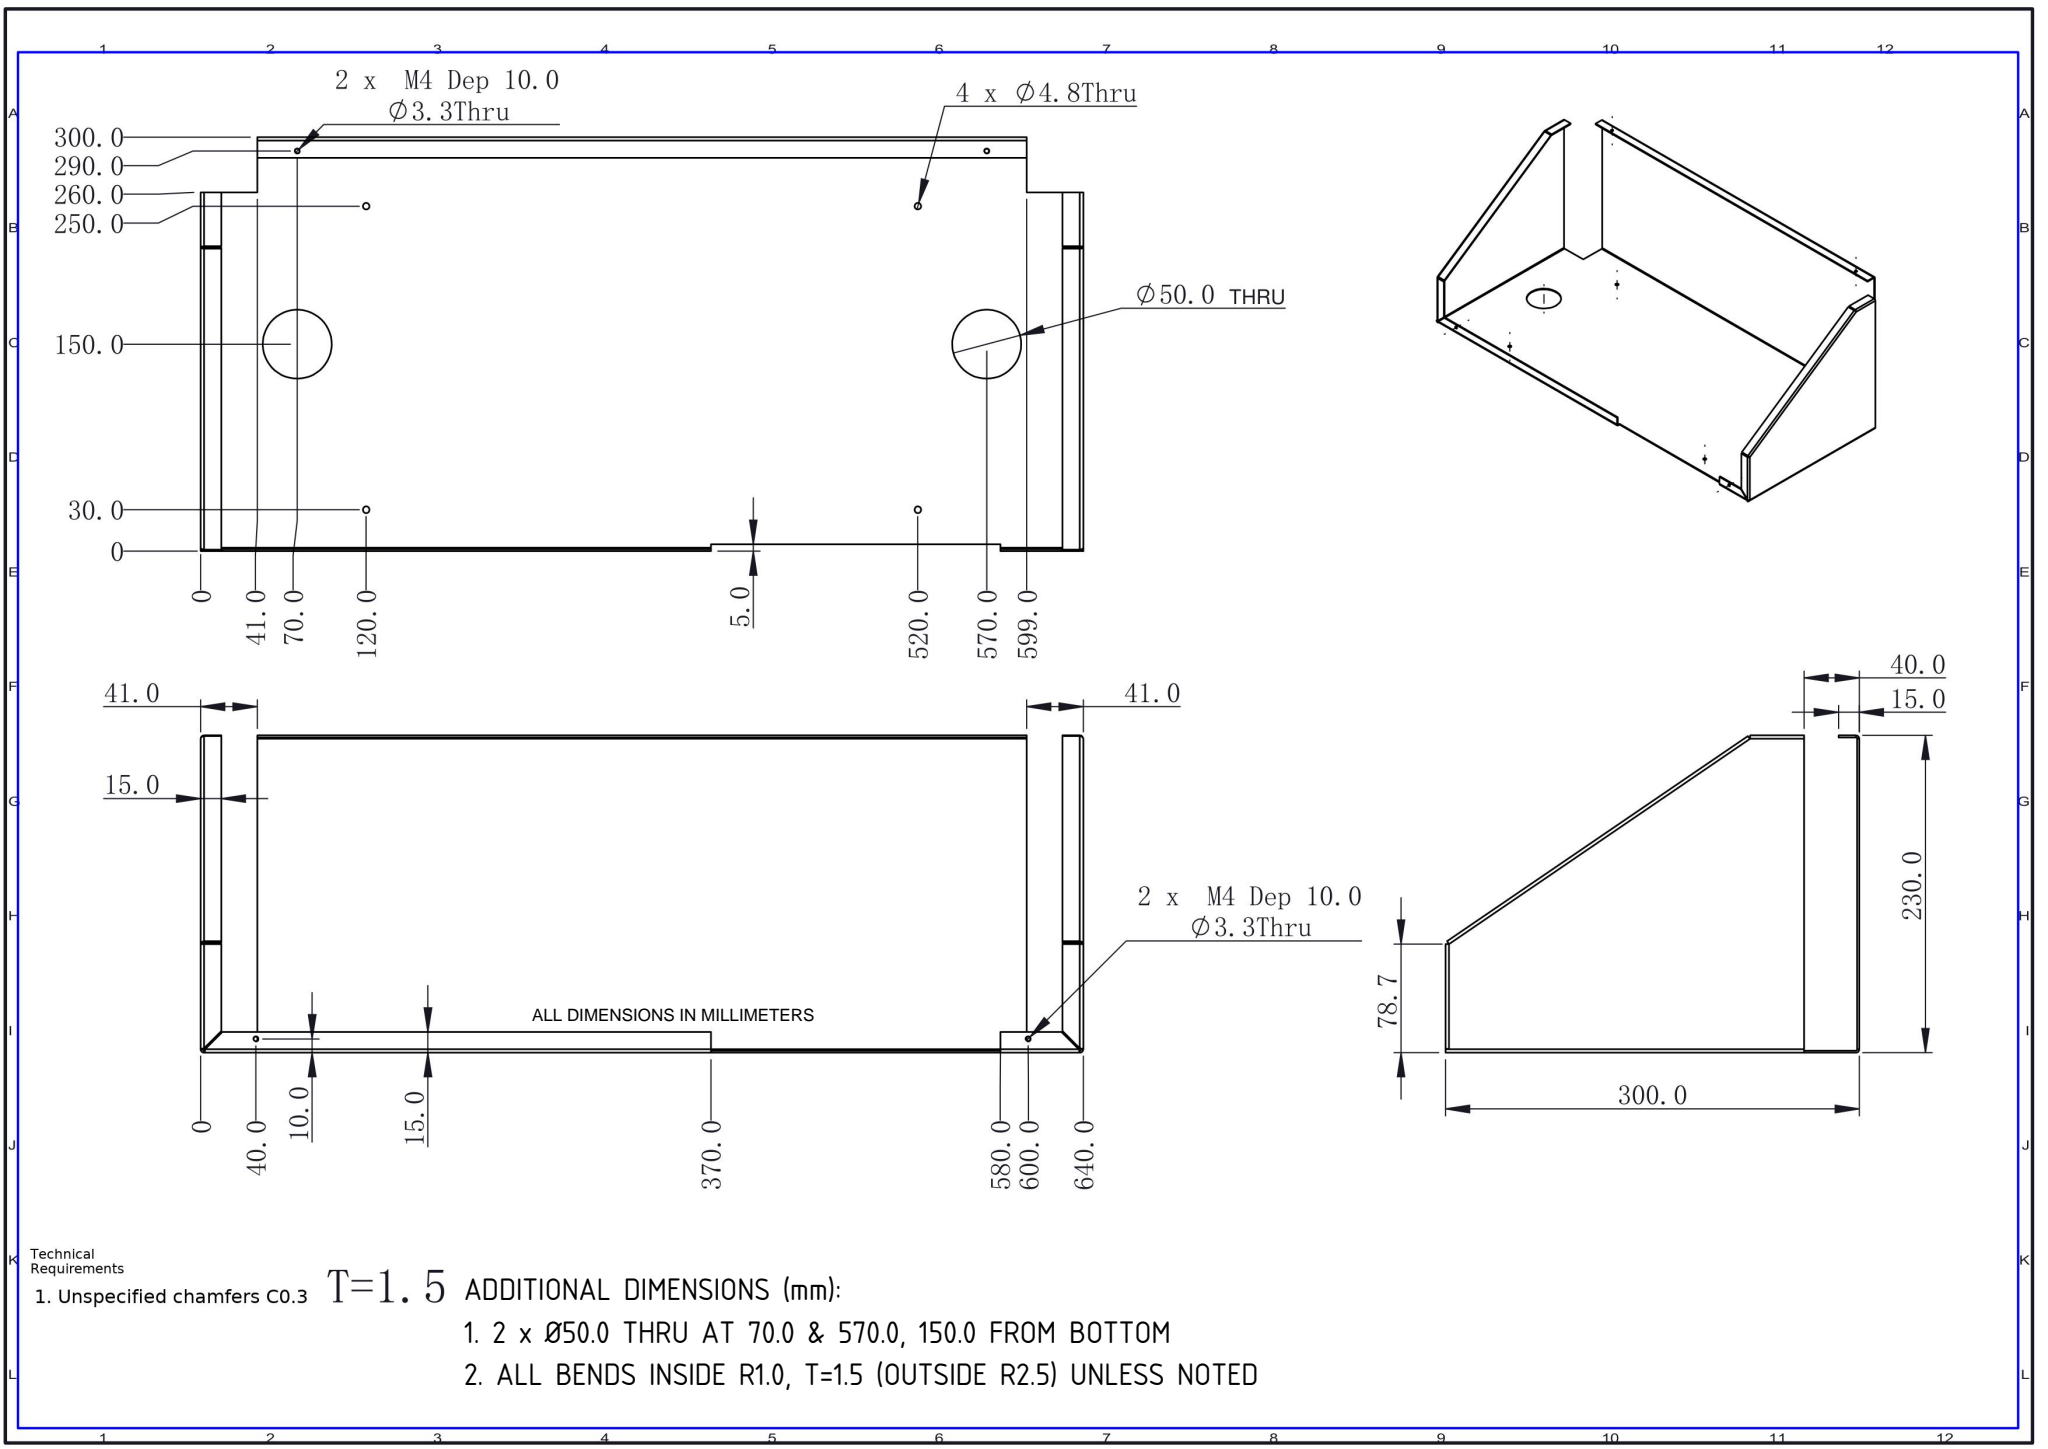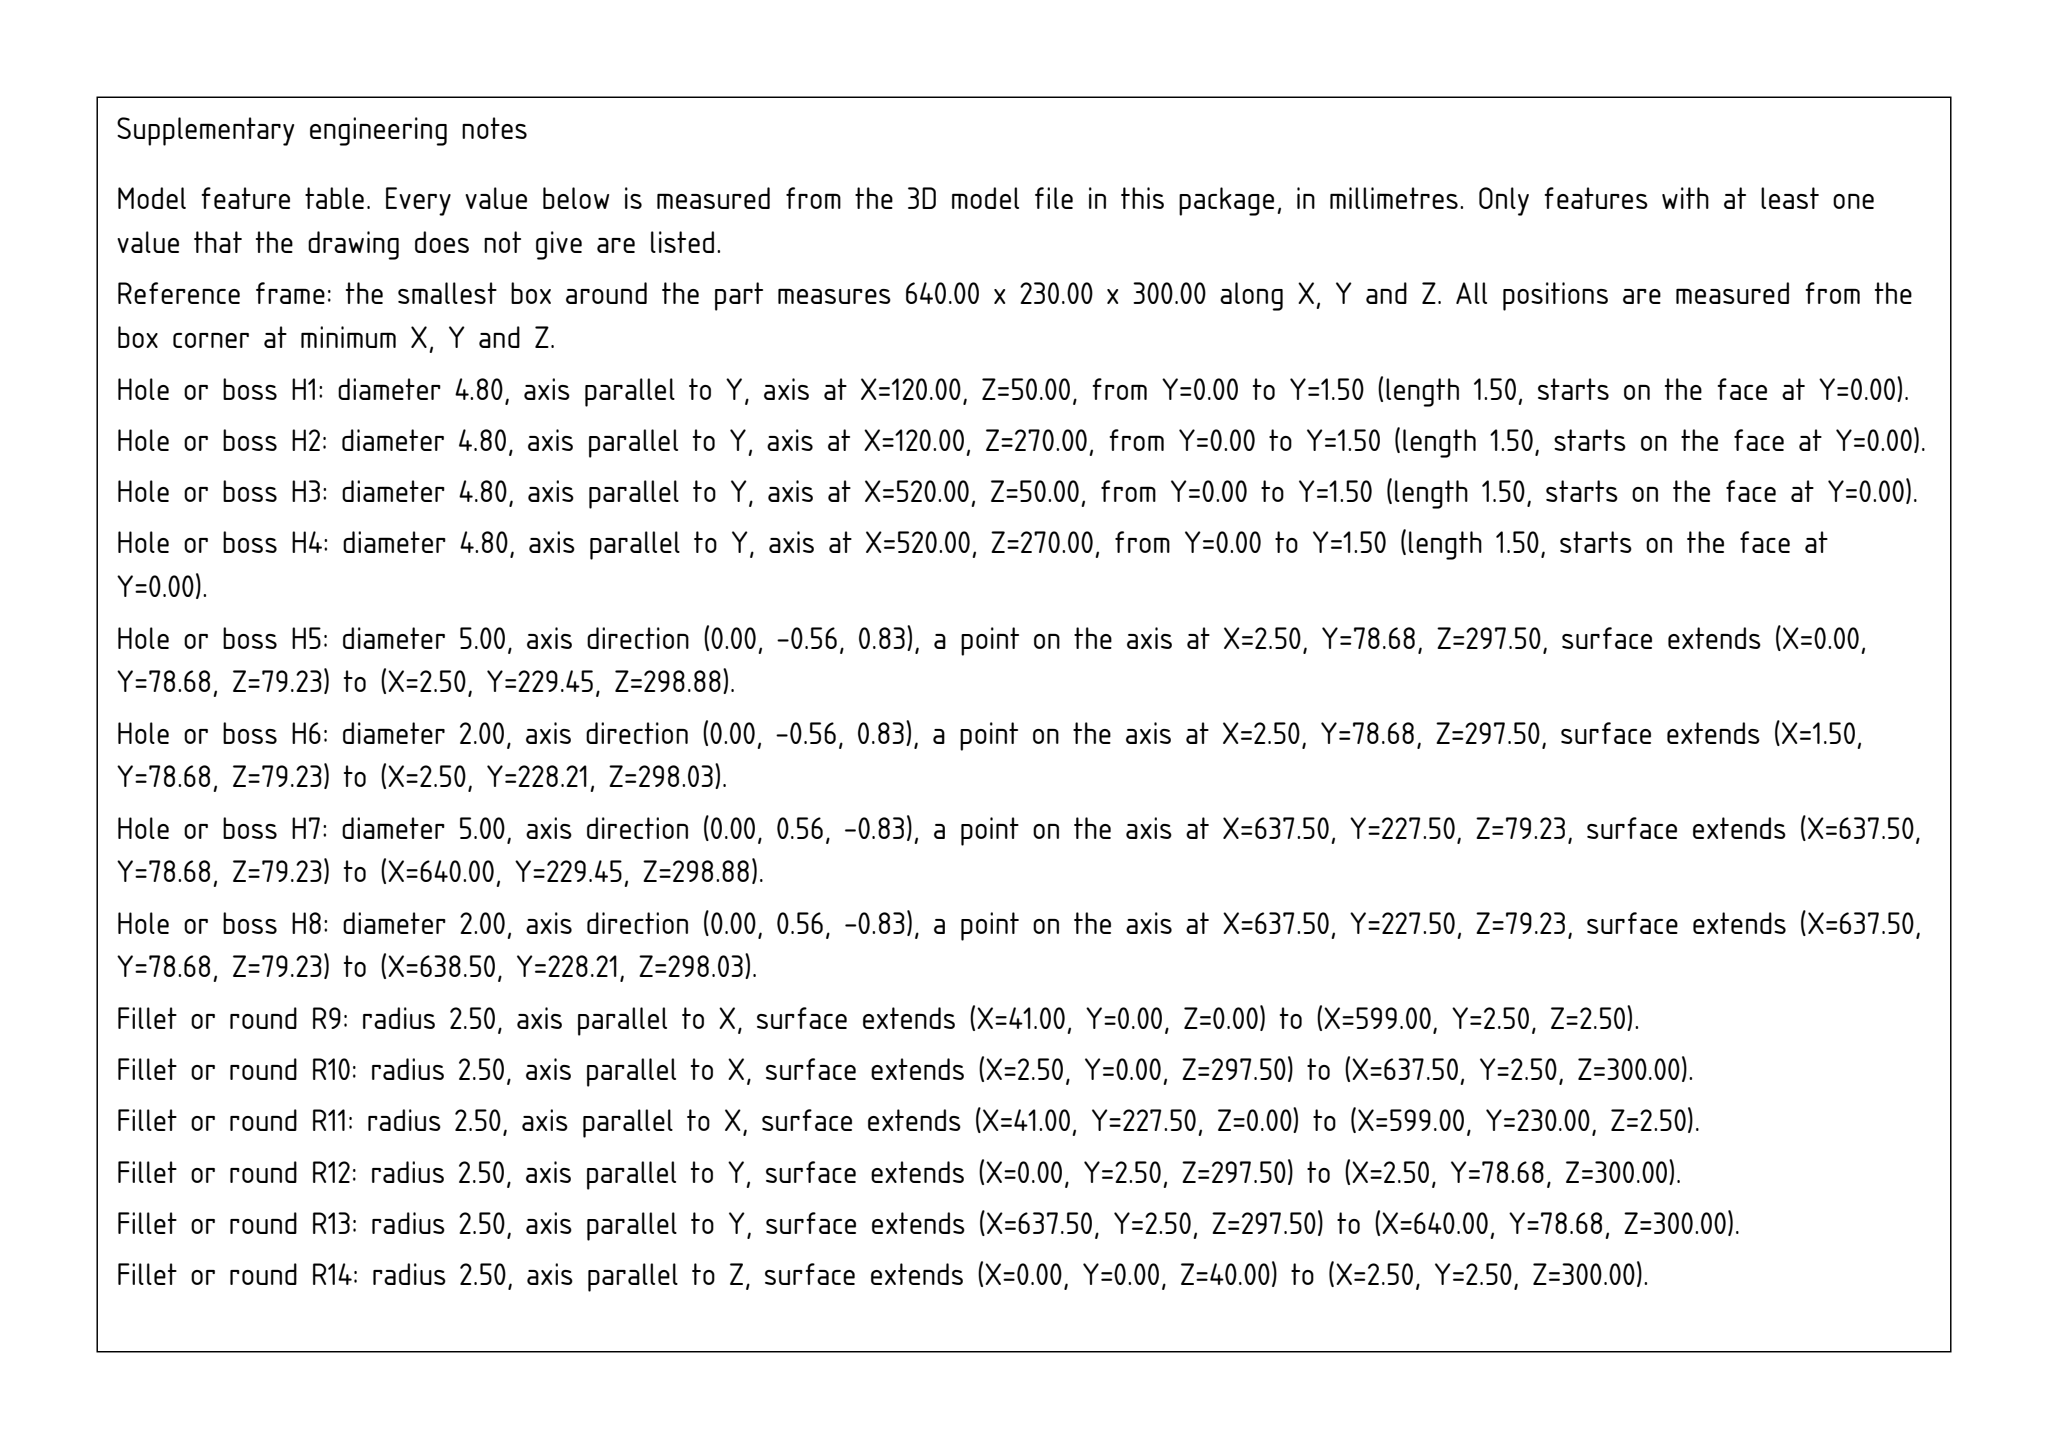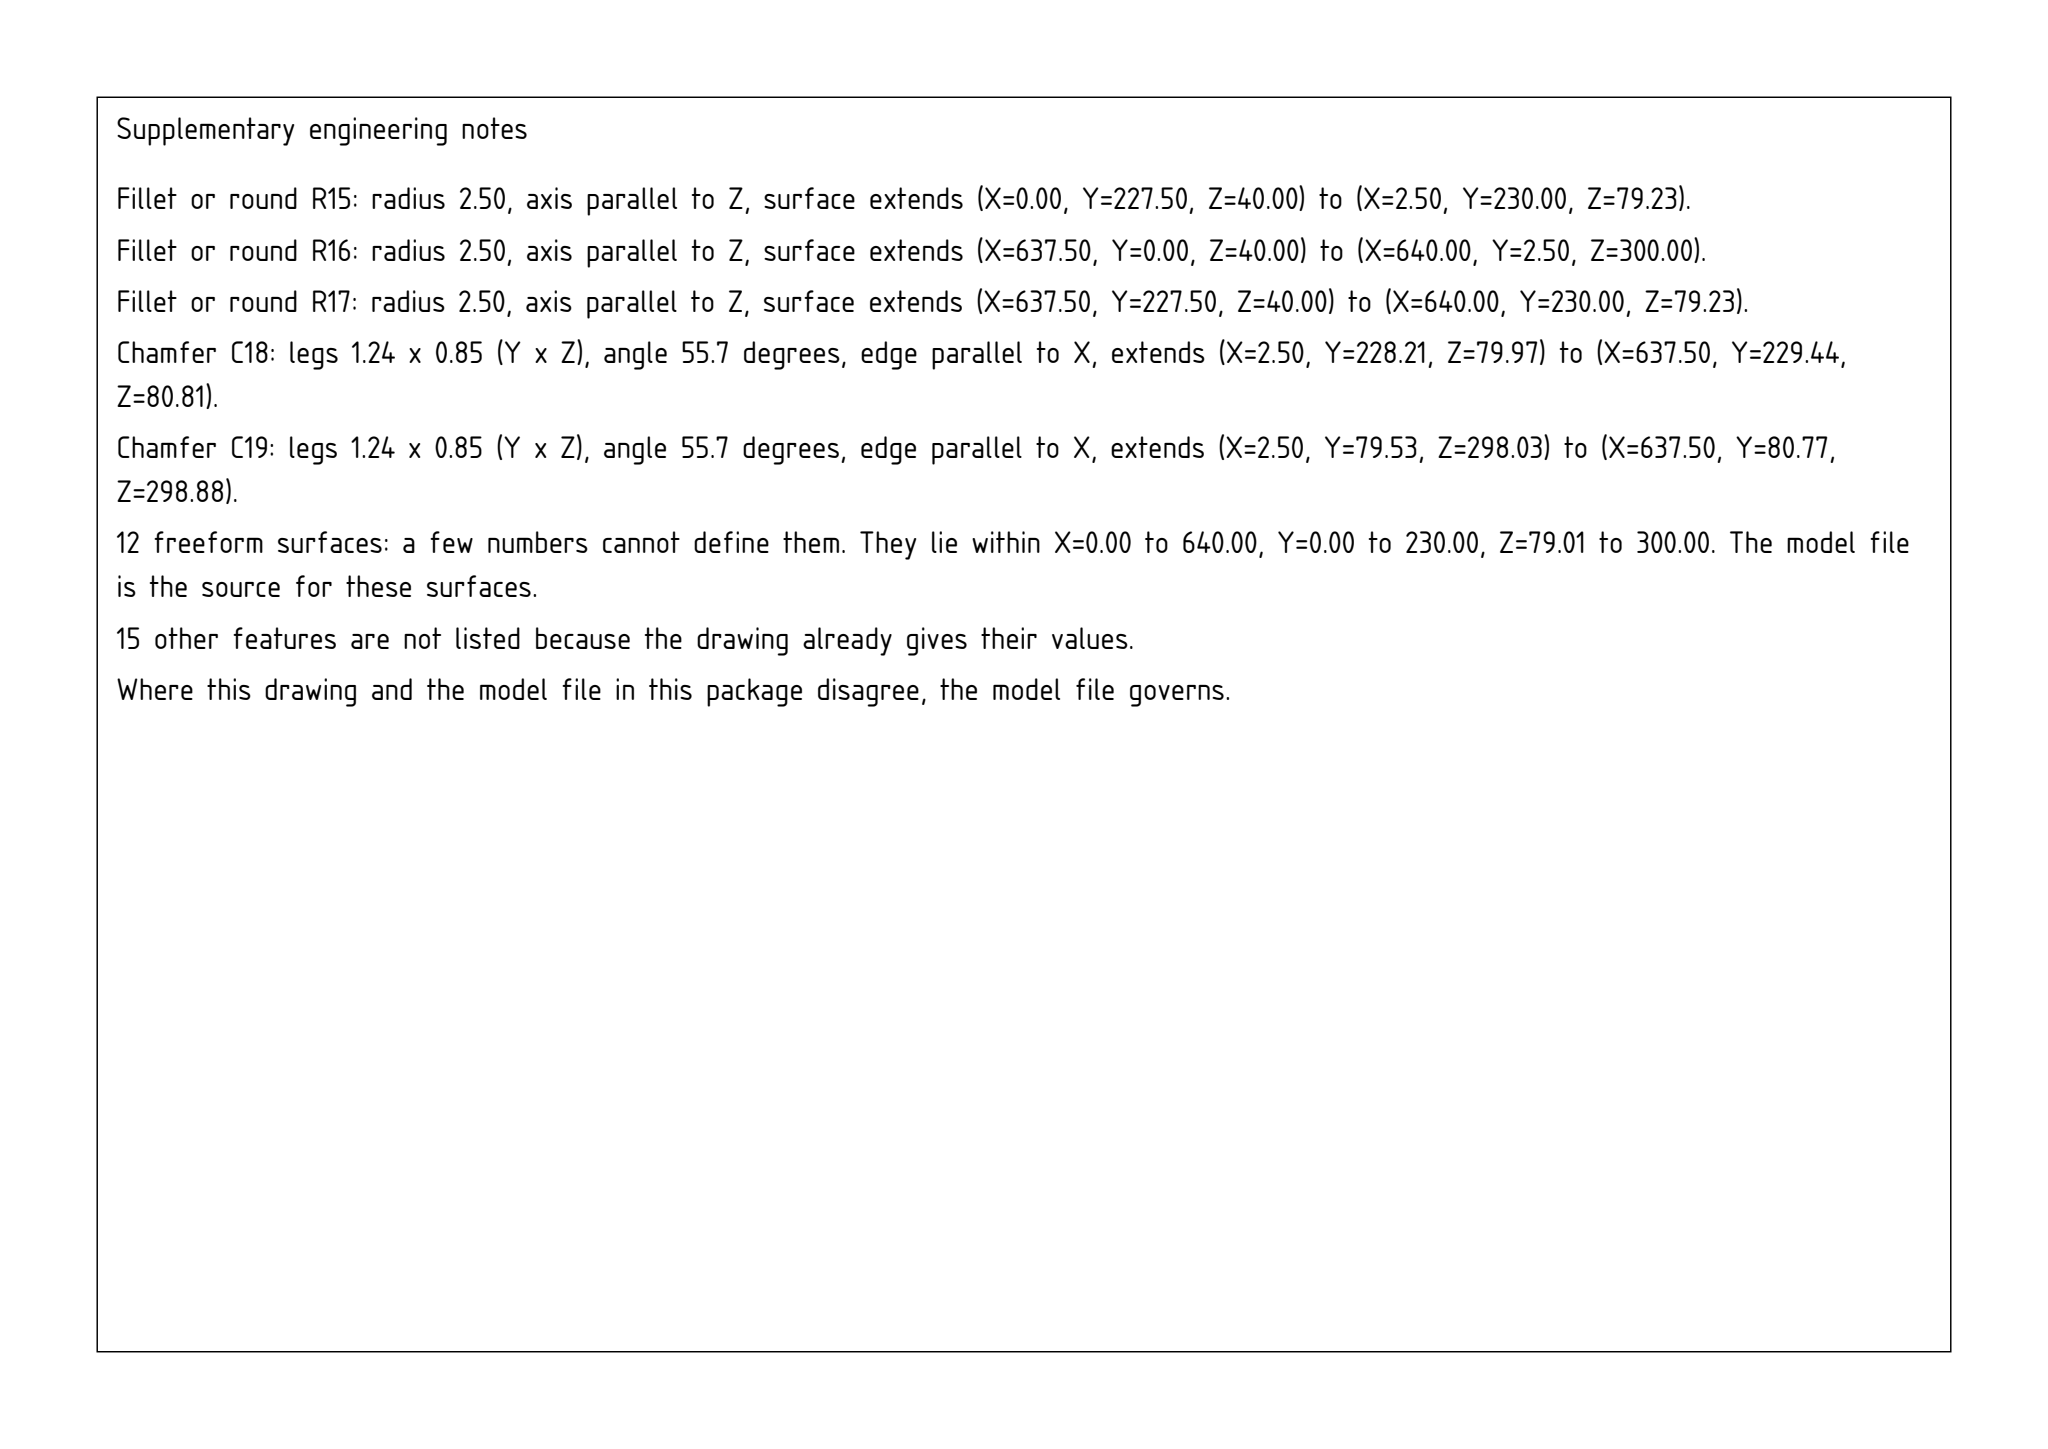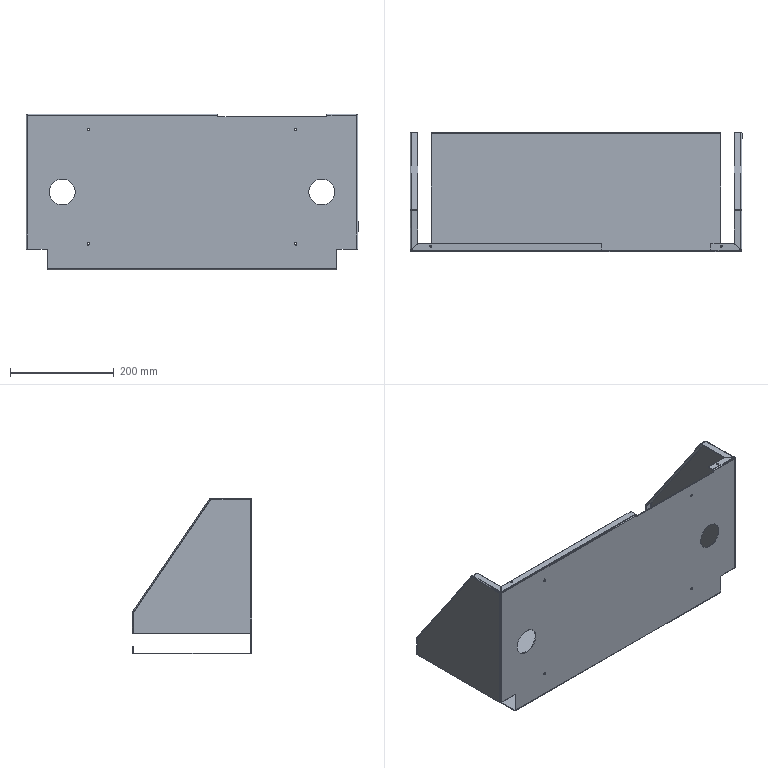Part | SolidWorks | mm | 1 solid | 128 faces | box 640 x 230 x 300 mm | volume 626976 mm3 | plane 72 | cylinder 44 | spline 12 | commonest cylinder face diameters 5 x12 2 x12 4.8 x8 3.3 x8 50 x4